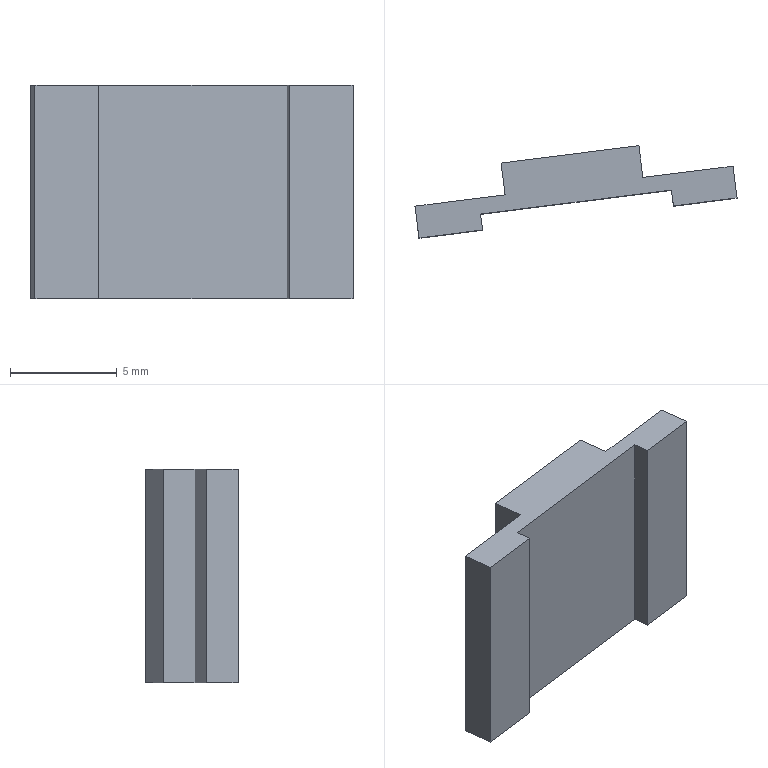Component | SolidWorks | BallJointRodUpperPressurePlate-1 | 1 solid | 14 faces | box 15.07 x 4.32 x 10 mm | volume 255 mm3 | plane 14
build123d program:
from build123d import *

# Parameters (mm, degrees)
SKETCH1_W           = 60
SKETCH1_H           = 40
BOSS_EXTRUDE1_DEPTH = 12
CUT_EXTRUDE1_DEPTH  = 52.42
SKETCH5_W           = 36
SKETCH5_H           = 6
CUT_EXTRUDE3_DEPTH  = 52.42
SCALE1_SCALE        = 0.25


with BuildPart() as part:
    # Sketch1 → Boss-Extrude1 (new body)
    with BuildSketch(Plane.XY):
        Rectangle(SKETCH1_W, SKETCH1_H)
    extrude(amount=BOSS_EXTRUDE1_DEPTH)

    # Sketch2 → Cut-Extrude1 (cut, through all)
    with BuildSketch(Plane(origin=(0, 20, 0), x_dir=(1, 0, 0), z_dir=(0, 1, 0))):
        Polygon((-30, -6), (-13, -6), (-13, 2.066), (13, 2.066), (13, -6), (30, -6), (30, 6.218), (-30, 6.961), align=None)
    extrude(amount=-CUT_EXTRUDE1_DEPTH, mode=Mode.SUBTRACT)

    # Sketch5 → Cut-Extrude3 (cut, through all)
    with BuildSketch(Plane(origin=(0, 20, 0), x_dir=(1, 0, 0), z_dir=(0, 1, 0))):
        with Locations((0, -12)):
            Rectangle(SKETCH5_W, SKETCH5_H)
    extrude(amount=-CUT_EXTRUDE3_DEPTH, mode=Mode.SUBTRACT)


with BuildPart() as part_1:
    # Scale1: scaled about (0, 0, 6.309)
    add(part.part.scale(SCALE1_SCALE).moved(Location((0, 0, 4.732))))


solid = part_1.part

# Placed as in the assembly
solid = solid.moved(Location((526.57, -310.68, 133.463), (90, 7.175, 0)))
STEP:
#1=CARTESIAN_POINT('',(21.062,-12.497,5.451));
#2=VERTEX_POINT('',#1);
#3=CARTESIAN_POINT('',(20.945,-12.511,5.451));
#4=VERTEX_POINT('',#3);
#5=CARTESIAN_POINT('',(20.476,-12.57,5.451));
#6=DIRECTION('',(-0.9922,-0.1249,-0.));
#7=VECTOR('',#6,39.37);
#8=LINE('',#5,#7);
#9=EDGE_CURVE('',#2,#4,#8,.T.);
#10=ORIENTED_EDGE('',*,*,#9,.T.);
#11=CARTESIAN_POINT('',(20.945,-12.511,5.058));
#12=VERTEX_POINT('',#11);
#13=CARTESIAN_POINT('',(20.945,-12.511,5.254));
#14=DIRECTION('',(0.,-0.,-1.));
#15=VECTOR('',#14,39.37);
#16=LINE('',#13,#15);
#17=EDGE_CURVE('',#4,#12,#16,.T.);
#18=ORIENTED_EDGE('',*,*,#17,.T.);
#19=CARTESIAN_POINT('',(21.062,-12.497,5.058));
#20=VERTEX_POINT('',#19);
#21=CARTESIAN_POINT('',(20.476,-12.57,5.058));
#22=DIRECTION('',(0.9922,0.1249,0.));
#23=VECTOR('',#22,39.37);
#24=LINE('',#21,#23);
#25=EDGE_CURVE('',#12,#20,#24,.T.);
#26=ORIENTED_EDGE('',*,*,#25,.T.);
#27=CARTESIAN_POINT('',(21.062,-12.497,5.058));
#28=DIRECTION('',(-0.,0.,1.));
#29=VECTOR('',#28,39.37);
#30=LINE('',#27,#29);
#31=EDGE_CURVE('',#20,#2,#30,.T.);
#32=ORIENTED_EDGE('',*,*,#31,.T.);
#33=EDGE_LOOP('',(#10,#18,#26,#32));
#34=FACE_OUTER_BOUND('',#33,.T.);
#35=CARTESIAN_POINT('',(20.769,-12.534,5.254));
#36=DIRECTION('',(-0.1249,0.9922,-0.));
#37=DIRECTION('',(-0.9922,-0.1249,-0.));
#38=AXIS2_PLACEMENT_3D('',#35,#36,#37);
#39=PLANE('',#38);
#40=ADVANCED_FACE('',(#34),#39,.F.);
#41=CARTESIAN_POINT('',(21.055,-12.438,5.058));
#42=VERTEX_POINT('',#41);
#43=CARTESIAN_POINT('',(21.062,-12.497,5.058));
#44=DIRECTION('',(-0.1249,0.9922,-0.));
#45=VECTOR('',#44,39.37);
#46=LINE('',#43,#45);
#47=EDGE_CURVE('',#20,#42,#46,.T.);
#48=ORIENTED_EDGE('',*,*,#47,.T.);
#49=CARTESIAN_POINT('',(21.055,-12.438,5.451));
#50=VERTEX_POINT('',#49);
#51=CARTESIAN_POINT('',(21.055,-12.438,5.058));
#52=DIRECTION('',(-0.,0.,1.));
#53=VECTOR('',#52,39.37);
#54=LINE('',#51,#53);
#55=EDGE_CURVE('',#42,#50,#54,.T.);
#56=ORIENTED_EDGE('',*,*,#55,.T.);
#57=CARTESIAN_POINT('',(21.062,-12.497,5.451));
#58=DIRECTION('',(-0.1249,0.9922,-0.));
#59=VECTOR('',#58,39.37);
#60=LINE('',#57,#59);
#61=EDGE_CURVE('',#2,#50,#60,.T.);
#62=ORIENTED_EDGE('',*,*,#61,.F.);
#63=ORIENTED_EDGE('',*,*,#31,.F.);
#64=EDGE_LOOP('',(#48,#56,#62,#63));
#65=FACE_OUTER_BOUND('',#64,.T.);
#66=CARTESIAN_POINT('',(21.062,-12.497,5.058));
#67=DIRECTION('',(-0.9922,-0.1249,-0.));
#68=DIRECTION('',(0.1249,-0.9922,0.));
#69=AXIS2_PLACEMENT_3D('',#66,#67,#68);
#70=PLANE('',#69);
#71=ADVANCED_FACE('',(#65),#70,.F.);
#72=CARTESIAN_POINT('',(20.941,-12.482,5.451));
#73=VERTEX_POINT('',#72);
#74=CARTESIAN_POINT('',(20.59,-12.526,5.451));
#75=VERTEX_POINT('',#74);
#76=CARTESIAN_POINT('',(20.59,-12.526,5.451));
#77=DIRECTION('',(-0.9922,-0.1249,-0.));
#78=VECTOR('',#77,39.37);
#79=LINE('',#76,#78);
#80=EDGE_CURVE('',#73,#75,#79,.T.);
#81=ORIENTED_EDGE('',*,*,#80,.F.);
#82=CARTESIAN_POINT('',(20.949,-12.541,5.451));
#83=DIRECTION('',(-0.1249,0.9922,-0.));
#84=VECTOR('',#83,39.37);
#85=LINE('',#82,#84);
#86=EDGE_CURVE('',#4,#73,#85,.T.);
#87=ORIENTED_EDGE('',*,*,#86,.F.);
#88=ORIENTED_EDGE('',*,*,#9,.F.);
#89=ORIENTED_EDGE('',*,*,#61,.T.);
#90=CARTESIAN_POINT('',(20.889,-12.459,5.451));
#91=VERTEX_POINT('',#90);
#92=CARTESIAN_POINT('',(20.889,-12.459,5.451));
#93=DIRECTION('',(0.9922,0.1249,0.));
#94=VECTOR('',#93,39.37);
#95=LINE('',#92,#94);
#96=EDGE_CURVE('',#91,#50,#95,.T.);
#97=ORIENTED_EDGE('',*,*,#96,.F.);
#98=CARTESIAN_POINT('',(20.881,-12.4,5.451));
#99=VERTEX_POINT('',#98);
#100=CARTESIAN_POINT('',(20.879,-12.38,5.451));
#101=DIRECTION('',(0.1249,-0.9922,0.));
#102=VECTOR('',#101,39.37);
#103=LINE('',#100,#102);
#104=EDGE_CURVE('',#99,#91,#103,.T.);
#105=ORIENTED_EDGE('',*,*,#104,.F.);
#106=CARTESIAN_POINT('',(20.627,-12.432,5.451));
#107=VERTEX_POINT('',#106);
#108=CARTESIAN_POINT('',(20.461,-12.453,5.451));
#109=DIRECTION('',(-0.9922,-0.1249,-0.));
#110=VECTOR('',#109,39.37);
#111=LINE('',#108,#110);
#112=EDGE_CURVE('',#99,#107,#111,.T.);
#113=ORIENTED_EDGE('',*,*,#112,.T.);
#114=CARTESIAN_POINT('',(20.635,-12.491,5.451));
#115=VERTEX_POINT('',#114);
#116=CARTESIAN_POINT('',(20.635,-12.491,5.451));
#117=DIRECTION('',(-0.1249,0.9922,-0.));
#118=VECTOR('',#117,39.37);
#119=LINE('',#116,#118);
#120=EDGE_CURVE('',#115,#107,#119,.T.);
#121=ORIENTED_EDGE('',*,*,#120,.F.);
#122=CARTESIAN_POINT('',(20.469,-12.512,5.451));
#123=VERTEX_POINT('',#122);
#124=CARTESIAN_POINT('',(20.469,-12.512,5.451));
#125=DIRECTION('',(0.9922,0.1249,0.));
#126=VECTOR('',#125,39.37);
#127=LINE('',#124,#126);
#128=EDGE_CURVE('',#123,#115,#127,.T.);
#129=ORIENTED_EDGE('',*,*,#128,.F.);
#130=CARTESIAN_POINT('',(20.476,-12.57,5.451));
#131=VERTEX_POINT('',#130);
#132=CARTESIAN_POINT('',(20.476,-12.57,5.451));
#133=DIRECTION('',(-0.1249,0.9922,-0.));
#134=VECTOR('',#133,39.37);
#135=LINE('',#132,#134);
#136=EDGE_CURVE('',#131,#123,#135,.T.);
#137=ORIENTED_EDGE('',*,*,#136,.F.);
#138=CARTESIAN_POINT('',(20.593,-12.556,5.451));
#139=VERTEX_POINT('',#138);
#140=CARTESIAN_POINT('',(20.476,-12.57,5.451));
#141=DIRECTION('',(-0.9922,-0.1249,-0.));
#142=VECTOR('',#141,39.37);
#143=LINE('',#140,#142);
#144=EDGE_CURVE('',#139,#131,#143,.T.);
#145=ORIENTED_EDGE('',*,*,#144,.F.);
#146=CARTESIAN_POINT('',(20.597,-12.585,5.451));
#147=DIRECTION('',(0.1249,-0.9922,0.));
#148=VECTOR('',#147,39.37);
#149=LINE('',#146,#148);
#150=EDGE_CURVE('',#75,#139,#149,.T.);
#151=ORIENTED_EDGE('',*,*,#150,.F.);
#152=EDGE_LOOP('',(#81,#87,#88,#89,#97,#105,#113,#121,#129,#137,#145,#151));
#153=FACE_OUTER_BOUND('',#152,.T.);
#154=CARTESIAN_POINT('',(20.476,-12.57,5.451));
#155=DIRECTION('',(0.,-0.,-1.));
#156=DIRECTION('',(-0.1249,0.9922,-0.));
#157=AXIS2_PLACEMENT_3D('',#154,#155,#156);
#158=PLANE('',#157);
#159=ADVANCED_FACE('',(#153),#158,.F.);
#160=ORIENTED_EDGE('',*,*,#136,.T.);
#161=CARTESIAN_POINT('',(20.469,-12.512,5.058));
#162=VERTEX_POINT('',#161);
#163=CARTESIAN_POINT('',(20.469,-12.512,5.058));
#164=DIRECTION('',(-0.,0.,1.));
#165=VECTOR('',#164,39.37);
#166=LINE('',#163,#165);
#167=EDGE_CURVE('',#162,#123,#166,.T.);
#168=ORIENTED_EDGE('',*,*,#167,.F.);
#169=CARTESIAN_POINT('',(20.476,-12.57,5.058));
#170=VERTEX_POINT('',#169);
#171=CARTESIAN_POINT('',(20.476,-12.57,5.058));
#172=DIRECTION('',(-0.1249,0.9922,-0.));
#173=VECTOR('',#172,39.37);
#174=LINE('',#171,#173);
#175=EDGE_CURVE('',#170,#162,#174,.T.);
#176=ORIENTED_EDGE('',*,*,#175,.F.);
#177=CARTESIAN_POINT('',(20.476,-12.57,5.058));
#178=DIRECTION('',(0.,-0.,-1.));
#179=VECTOR('',#178,39.37);
#180=LINE('',#177,#179);
#181=EDGE_CURVE('',#131,#170,#180,.T.);
#182=ORIENTED_EDGE('',*,*,#181,.F.);
#183=EDGE_LOOP('',(#160,#168,#176,#182));
#184=FACE_OUTER_BOUND('',#183,.T.);
#185=CARTESIAN_POINT('',(20.476,-12.57,5.058));
#186=DIRECTION('',(0.9922,0.1249,0.));
#187=DIRECTION('',(-0.1249,0.9922,-0.));
#188=AXIS2_PLACEMENT_3D('',#185,#186,#187);
#189=PLANE('',#188);
#190=ADVANCED_FACE('',(#184),#189,.F.);
#191=ORIENTED_EDGE('',*,*,#25,.F.);
#192=CARTESIAN_POINT('',(20.941,-12.482,5.058));
#193=VERTEX_POINT('',#192);
#194=CARTESIAN_POINT('',(20.949,-12.541,5.058));
#195=DIRECTION('',(-0.1249,0.9922,-0.));
#196=VECTOR('',#195,39.37);
#197=LINE('',#194,#196);
#198=EDGE_CURVE('',#12,#193,#197,.T.);
#199=ORIENTED_EDGE('',*,*,#198,.T.);
#200=CARTESIAN_POINT('',(20.59,-12.526,5.058));
#201=VERTEX_POINT('',#200);
#202=CARTESIAN_POINT('',(20.59,-12.526,5.058));
#203=DIRECTION('',(-0.9922,-0.1249,-0.));
#204=VECTOR('',#203,39.37);
#205=LINE('',#202,#204);
#206=EDGE_CURVE('',#193,#201,#205,.T.);
#207=ORIENTED_EDGE('',*,*,#206,.T.);
#208=CARTESIAN_POINT('',(20.593,-12.556,5.058));
#209=VERTEX_POINT('',#208);
#210=CARTESIAN_POINT('',(20.597,-12.585,5.058));
#211=DIRECTION('',(0.1249,-0.9922,0.));
#212=VECTOR('',#211,39.37);
#213=LINE('',#210,#212);
#214=EDGE_CURVE('',#201,#209,#213,.T.);
#215=ORIENTED_EDGE('',*,*,#214,.T.);
#216=CARTESIAN_POINT('',(20.476,-12.57,5.058));
#217=DIRECTION('',(0.9922,0.1249,0.));
#218=VECTOR('',#217,39.37);
#219=LINE('',#216,#218);
#220=EDGE_CURVE('',#170,#209,#219,.T.);
#221=ORIENTED_EDGE('',*,*,#220,.F.);
#222=ORIENTED_EDGE('',*,*,#175,.T.);
#223=CARTESIAN_POINT('',(20.635,-12.491,5.058));
#224=VERTEX_POINT('',#223);
#225=CARTESIAN_POINT('',(20.469,-12.512,5.058));
#226=DIRECTION('',(0.9922,0.1249,0.));
#227=VECTOR('',#226,39.37);
#228=LINE('',#225,#227);
#229=EDGE_CURVE('',#162,#224,#228,.T.);
#230=ORIENTED_EDGE('',*,*,#229,.T.);
#231=CARTESIAN_POINT('',(20.627,-12.432,5.058));
#232=VERTEX_POINT('',#231);
#233=CARTESIAN_POINT('',(20.635,-12.491,5.058));
#234=DIRECTION('',(-0.1249,0.9922,-0.));
#235=VECTOR('',#234,39.37);
#236=LINE('',#233,#235);
#237=EDGE_CURVE('',#224,#232,#236,.T.);
#238=ORIENTED_EDGE('',*,*,#237,.T.);
#239=CARTESIAN_POINT('',(20.881,-12.4,5.058));
#240=VERTEX_POINT('',#239);
#241=CARTESIAN_POINT('',(20.461,-12.453,5.058));
#242=DIRECTION('',(0.9922,0.1249,0.));
#243=VECTOR('',#242,39.37);
#244=LINE('',#241,#243);
#245=EDGE_CURVE('',#232,#240,#244,.T.);
#246=ORIENTED_EDGE('',*,*,#245,.T.);
#247=CARTESIAN_POINT('',(20.889,-12.459,5.058));
#248=VERTEX_POINT('',#247);
#249=CARTESIAN_POINT('',(20.879,-12.38,5.058));
#250=DIRECTION('',(0.1249,-0.9922,0.));
#251=VECTOR('',#250,39.37);
#252=LINE('',#249,#251);
#253=EDGE_CURVE('',#240,#248,#252,.T.);
#254=ORIENTED_EDGE('',*,*,#253,.T.);
#255=CARTESIAN_POINT('',(20.889,-12.459,5.058));
#256=DIRECTION('',(0.9922,0.1249,0.));
#257=VECTOR('',#256,39.37);
#258=LINE('',#255,#257);
#259=EDGE_CURVE('',#248,#42,#258,.T.);
#260=ORIENTED_EDGE('',*,*,#259,.T.);
#261=ORIENTED_EDGE('',*,*,#47,.F.);
#262=EDGE_LOOP('',(#191,#199,#207,#215,#221,#222,#230,#238,#246,#254,#260,#261));
#263=FACE_OUTER_BOUND('',#262,.T.);
#264=CARTESIAN_POINT('',(20.476,-12.57,5.058));
#265=DIRECTION('',(-0.,0.,1.));
#266=DIRECTION('',(0.1249,-0.9922,0.));
#267=AXIS2_PLACEMENT_3D('',#264,#265,#266);
#268=PLANE('',#267);
#269=ADVANCED_FACE('',(#263),#268,.F.);
#270=ORIENTED_EDGE('',*,*,#220,.T.);
#271=CARTESIAN_POINT('',(20.593,-12.556,5.254));
#272=DIRECTION('',(-0.,0.,1.));
#273=VECTOR('',#272,39.37);
#274=LINE('',#271,#273);
#275=EDGE_CURVE('',#209,#139,#274,.T.);
#276=ORIENTED_EDGE('',*,*,#275,.T.);
#277=ORIENTED_EDGE('',*,*,#144,.T.);
#278=ORIENTED_EDGE('',*,*,#181,.T.);
#279=EDGE_LOOP('',(#270,#276,#277,#278));
#280=FACE_OUTER_BOUND('',#279,.T.);
#281=CARTESIAN_POINT('',(20.769,-12.534,5.254));
#282=DIRECTION('',(-0.1249,0.9922,-0.));
#283=DIRECTION('',(-0.9922,-0.1249,-0.));
#284=AXIS2_PLACEMENT_3D('',#281,#282,#283);
#285=PLANE('',#284);
#286=ADVANCED_FACE('',(#280),#285,.F.);
#287=CARTESIAN_POINT('',(20.881,-12.4,5.254));
#288=DIRECTION('',(-0.,0.,1.));
#289=VECTOR('',#288,39.37);
#290=LINE('',#287,#289);
#291=EDGE_CURVE('',#240,#99,#290,.T.);
#292=ORIENTED_EDGE('',*,*,#291,.F.);
#293=ORIENTED_EDGE('',*,*,#245,.F.);
#294=CARTESIAN_POINT('',(20.627,-12.432,5.254));
#295=DIRECTION('',(0.,-0.,-1.));
#296=VECTOR('',#295,39.37);
#297=LINE('',#294,#296);
#298=EDGE_CURVE('',#107,#232,#297,.T.);
#299=ORIENTED_EDGE('',*,*,#298,.F.);
#300=ORIENTED_EDGE('',*,*,#112,.F.);
#301=EDGE_LOOP('',(#292,#293,#299,#300));
#302=FACE_OUTER_BOUND('',#301,.T.);
#303=CARTESIAN_POINT('',(20.754,-12.416,5.254));
#304=DIRECTION('',(-0.1249,0.9922,-0.));
#305=DIRECTION('',(-0.9922,-0.1249,-0.));
#306=AXIS2_PLACEMENT_3D('',#303,#304,#305);
#307=PLANE('',#306);
#308=ADVANCED_FACE('',(#302),#307,.T.);
#309=ORIENTED_EDGE('',*,*,#298,.T.);
#310=ORIENTED_EDGE('',*,*,#237,.F.);
#311=CARTESIAN_POINT('',(20.635,-12.491,5.058));
#312=DIRECTION('',(-0.,0.,1.));
#313=VECTOR('',#312,39.37);
#314=LINE('',#311,#313);
#315=EDGE_CURVE('',#224,#115,#314,.T.);
#316=ORIENTED_EDGE('',*,*,#315,.T.);
#317=ORIENTED_EDGE('',*,*,#120,.T.);
#318=EDGE_LOOP('',(#309,#310,#316,#317));
#319=FACE_OUTER_BOUND('',#318,.T.);
#320=CARTESIAN_POINT('',(20.635,-12.491,5.058));
#321=DIRECTION('',(0.9922,0.1249,0.));
#322=DIRECTION('',(-0.1249,0.9922,-0.));
#323=AXIS2_PLACEMENT_3D('',#320,#321,#322);
#324=PLANE('',#323);
#325=ADVANCED_FACE('',(#319),#324,.F.);
#326=ORIENTED_EDGE('',*,*,#128,.T.);
#327=ORIENTED_EDGE('',*,*,#315,.F.);
#328=ORIENTED_EDGE('',*,*,#229,.F.);
#329=ORIENTED_EDGE('',*,*,#167,.T.);
#330=EDGE_LOOP('',(#326,#327,#328,#329));
#331=FACE_OUTER_BOUND('',#330,.T.);
#332=CARTESIAN_POINT('',(20.469,-12.512,5.058));
#333=DIRECTION('',(0.1249,-0.9922,0.));
#334=DIRECTION('',(0.9922,0.1249,0.));
#335=AXIS2_PLACEMENT_3D('',#332,#333,#334);
#336=PLANE('',#335);
#337=ADVANCED_FACE('',(#331),#336,.F.);
#338=ORIENTED_EDGE('',*,*,#96,.T.);
#339=ORIENTED_EDGE('',*,*,#55,.F.);
#340=ORIENTED_EDGE('',*,*,#259,.F.);
#341=CARTESIAN_POINT('',(20.889,-12.459,5.058));
#342=DIRECTION('',(-0.,0.,1.));
#343=VECTOR('',#342,39.37);
#344=LINE('',#341,#343);
#345=EDGE_CURVE('',#248,#91,#344,.T.);
#346=ORIENTED_EDGE('',*,*,#345,.T.);
#347=EDGE_LOOP('',(#338,#339,#340,#346));
#348=FACE_OUTER_BOUND('',#347,.T.);
#349=CARTESIAN_POINT('',(20.889,-12.459,5.058));
#350=DIRECTION('',(0.1249,-0.9922,0.));
#351=DIRECTION('',(0.9922,0.1249,0.));
#352=AXIS2_PLACEMENT_3D('',#349,#350,#351);
#353=PLANE('',#352);
#354=ADVANCED_FACE('',(#348),#353,.F.);
#355=ORIENTED_EDGE('',*,*,#291,.T.);
#356=ORIENTED_EDGE('',*,*,#104,.T.);
#357=ORIENTED_EDGE('',*,*,#345,.F.);
#358=ORIENTED_EDGE('',*,*,#253,.F.);
#359=EDGE_LOOP('',(#355,#356,#357,#358));
#360=FACE_OUTER_BOUND('',#359,.T.);
#361=CARTESIAN_POINT('',(20.879,-12.38,5.058));
#362=DIRECTION('',(-0.9922,-0.1249,-0.));
#363=DIRECTION('',(0.1249,-0.9922,0.));
#364=AXIS2_PLACEMENT_3D('',#361,#362,#363);
#365=PLANE('',#364);
#366=ADVANCED_FACE('',(#360),#365,.F.);
#367=ORIENTED_EDGE('',*,*,#86,.T.);
#368=CARTESIAN_POINT('',(20.941,-12.482,5.058));
#369=DIRECTION('',(-0.,0.,1.));
#370=VECTOR('',#369,39.37);
#371=LINE('',#368,#370);
#372=EDGE_CURVE('',#193,#73,#371,.T.);
#373=ORIENTED_EDGE('',*,*,#372,.F.);
#374=ORIENTED_EDGE('',*,*,#198,.F.);
#375=ORIENTED_EDGE('',*,*,#17,.F.);
#376=EDGE_LOOP('',(#367,#373,#374,#375));
#377=FACE_OUTER_BOUND('',#376,.T.);
#378=CARTESIAN_POINT('',(20.949,-12.541,5.058));
#379=DIRECTION('',(0.9922,0.1249,0.));
#380=DIRECTION('',(-0.1249,0.9922,-0.));
#381=AXIS2_PLACEMENT_3D('',#378,#379,#380);
#382=PLANE('',#381);
#383=ADVANCED_FACE('',(#377),#382,.F.);
#384=ORIENTED_EDGE('',*,*,#214,.F.);
#385=CARTESIAN_POINT('',(20.59,-12.526,5.058));
#386=DIRECTION('',(-0.,0.,1.));
#387=VECTOR('',#386,39.37);
#388=LINE('',#385,#387);
#389=EDGE_CURVE('',#201,#75,#388,.T.);
#390=ORIENTED_EDGE('',*,*,#389,.T.);
#391=ORIENTED_EDGE('',*,*,#150,.T.);
#392=ORIENTED_EDGE('',*,*,#275,.F.);
#393=EDGE_LOOP('',(#384,#390,#391,#392));
#394=FACE_OUTER_BOUND('',#393,.T.);
#395=CARTESIAN_POINT('',(20.597,-12.585,5.058));
#396=DIRECTION('',(-0.9922,-0.1249,-0.));
#397=DIRECTION('',(0.1249,-0.9922,0.));
#398=AXIS2_PLACEMENT_3D('',#395,#396,#397);
#399=PLANE('',#398);
#400=ADVANCED_FACE('',(#394),#399,.F.);
#401=ORIENTED_EDGE('',*,*,#80,.T.);
#402=ORIENTED_EDGE('',*,*,#389,.F.);
#403=ORIENTED_EDGE('',*,*,#206,.F.);
#404=ORIENTED_EDGE('',*,*,#372,.T.);
#405=EDGE_LOOP('',(#401,#402,#403,#404));
#406=FACE_OUTER_BOUND('',#405,.T.);
#407=CARTESIAN_POINT('',(20.59,-12.526,5.058));
#408=DIRECTION('',(-0.1249,0.9922,-0.));
#409=DIRECTION('',(-0.9922,-0.1249,-0.));
#410=AXIS2_PLACEMENT_3D('',#407,#408,#409);
#411=PLANE('',#410);
#412=ADVANCED_FACE('',(#406),#411,.F.);
#413=CLOSED_SHELL('',(#40,#71,#159,#190,#269,#286,#308,#325,#337,#354,#366,#383,#400,#412));
#414=MANIFOLD_SOLID_BREP('',#413);
#415=CARTESIAN_POINT('',(0.,0.,0.));
#416=DIRECTION('',(0.,0.,1.));
#417=DIRECTION('',(1.,0.,0.));
#418=AXIS2_PLACEMENT_3D('',#415,#416,#417);
#419=(LENGTH_UNIT()NAMED_UNIT(*)SI_UNIT($,.METRE.));
#420=LENGTH_MEASURE_WITH_UNIT(LENGTH_MEASURE(0.0254),#419);
#421=DIMENSIONAL_EXPONENTS(1.,0.,0.,0.,0.,0.,0.);
#422=(CONVERSION_BASED_UNIT('',#420)LENGTH_UNIT()NAMED_UNIT(#421));
#423=UNCERTAINTY_MEASURE_WITH_UNIT(LENGTH_MEASURE(0.00001),#422,'','');
#424=(NAMED_UNIT(*)PLANE_ANGLE_UNIT()SI_UNIT($,.RADIAN.));
#425=(NAMED_UNIT(*)SI_UNIT($,.STERADIAN.)SOLID_ANGLE_UNIT());
#426=(GEOMETRIC_REPRESENTATION_CONTEXT(3)GLOBAL_UNCERTAINTY_ASSIGNED_CONTEXT((#423))GLOBAL_UNIT_ASSIGNED_CONTEXT((#422,#424,#425))REPRESENTATION_CONTEXT('',''));
#427=ADVANCED_BREP_SHAPE_REPRESENTATION('',(#414,#418),#426);
#428=COLOUR_RGB('',0.7922,0.8196,0.9333);
#429=FILL_AREA_STYLE_COLOUR('',#428);
#430=FILL_AREA_STYLE('',(#429));
#431=SURFACE_STYLE_FILL_AREA(#430);
#432=SURFACE_SIDE_STYLE('',(#431));
#433=SURFACE_STYLE_USAGE(.BOTH.,#432);
#434=PRESENTATION_STYLE_ASSIGNMENT((#433));
#435=STYLED_ITEM('',(#434),#414);
#436=(LENGTH_UNIT()NAMED_UNIT(*)SI_UNIT($,.METRE.));
#437=LENGTH_MEASURE_WITH_UNIT(LENGTH_MEASURE(0.0254),#436);
#438=DIMENSIONAL_EXPONENTS(1.,0.,0.,0.,0.,0.,0.);
#439=(CONVERSION_BASED_UNIT('',#437)LENGTH_UNIT()NAMED_UNIT(#438));
#440=UNCERTAINTY_MEASURE_WITH_UNIT(LENGTH_MEASURE(0.00001),#439,'','');
#441=(NAMED_UNIT(*)PLANE_ANGLE_UNIT()SI_UNIT($,.RADIAN.));
#442=(NAMED_UNIT(*)SI_UNIT($,.STERADIAN.)SOLID_ANGLE_UNIT());
#443=(GEOMETRIC_REPRESENTATION_CONTEXT(3)GLOBAL_UNCERTAINTY_ASSIGNED_CONTEXT((#440))GLOBAL_UNIT_ASSIGNED_CONTEXT((#439,#441,#442))REPRESENTATION_CONTEXT('',''));
#444=MECHANICAL_DESIGN_GEOMETRIC_PRESENTATION_REPRESENTATION('',(#435),#443);
#445=PRESENTATION_LAYER_ASSIGNMENT('','',(#435));